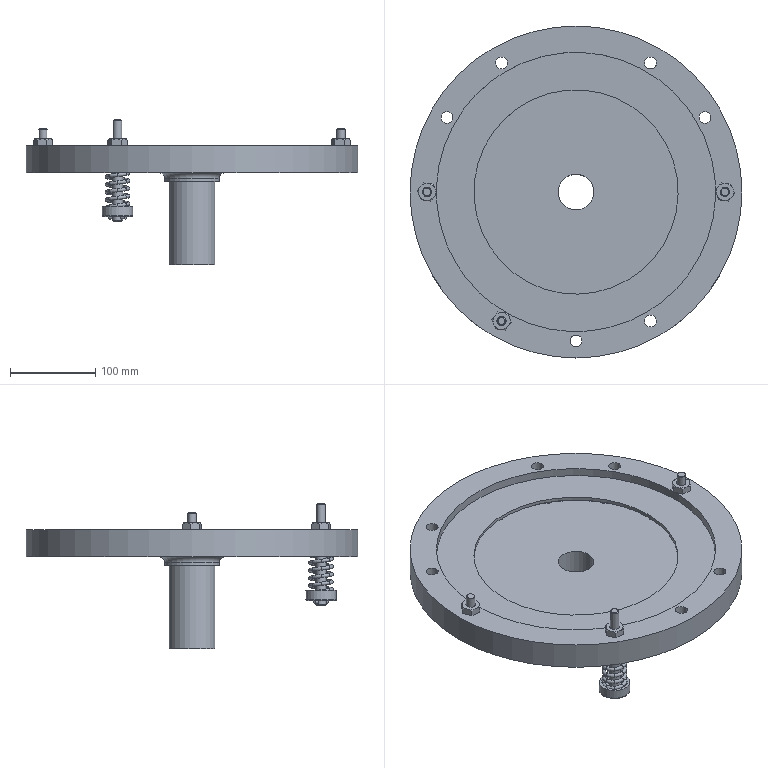Assembly | NX | mm | 9 component files | 10 solids | 213 faces | box 390 x 390 x 171.17 mm | volume 2638499 mm3 | plane 71 | cylinder 52 | torus 50 | cone 40 | commonest cylinder face diameters 3 x12 11 x9 14 x9 30 x7 10 x3 3.2 x2 36 x1 12.5 x1
Bill of materials:
unnamed part 1 | 3 |  | Hexagonal prism with a central cylindrical through-bore and a conical chamfer on the corners of one face; looks like a hex nut.
unnamed part 2 | 1 |  | Cylindrical helical coil of round-section wire with constant coil diameter and evenly spaced open turns, about 6-7 turns.
unnamed part 3 | 1 |  | Stepped cylindrical pin with a smaller-diameter upper section and a longer larger-diameter lower section; a small cross pin passes through near the bottom end and sticks out on both sides.
unnamed part 4 | 2 |  | Hex-headed fastener-like part: a plain cylindrical shank on a hexagonal head, with a chamfered shank tip and a chamfered head edge on the side away from the shank.
unnamed part 5 | 1 |  | Flat circular disc flange with a ring of small through-holes near the edge, a central through-hole, two concentric shallow circular grooves or steps on the top face, and a cylindrical tubular stem under the center.
unnamed part 6 | 1 |  | Short thick-walled cylindrical cup or ring with a large counterbore from one face and a smaller central through-hole in the floor, plus a small rounded edge on the outer bottom.
Mates:
1. fix | Driven_Flange 1 component
2. concentric | HexScrewM10 1 edge | Driven_Flange 1 edge
3. concentric | HexnutM12 2 edge | Driven_Flange 1 edge
4. concentric | HexScrewM10 2 edge | Driven_Flange 1 edge
5. concentric | HexnutM12 3 edge | Driven_Flange 1 edge
6. concentric | HexnutM12 1 edge | Driven_Flange 1 edge